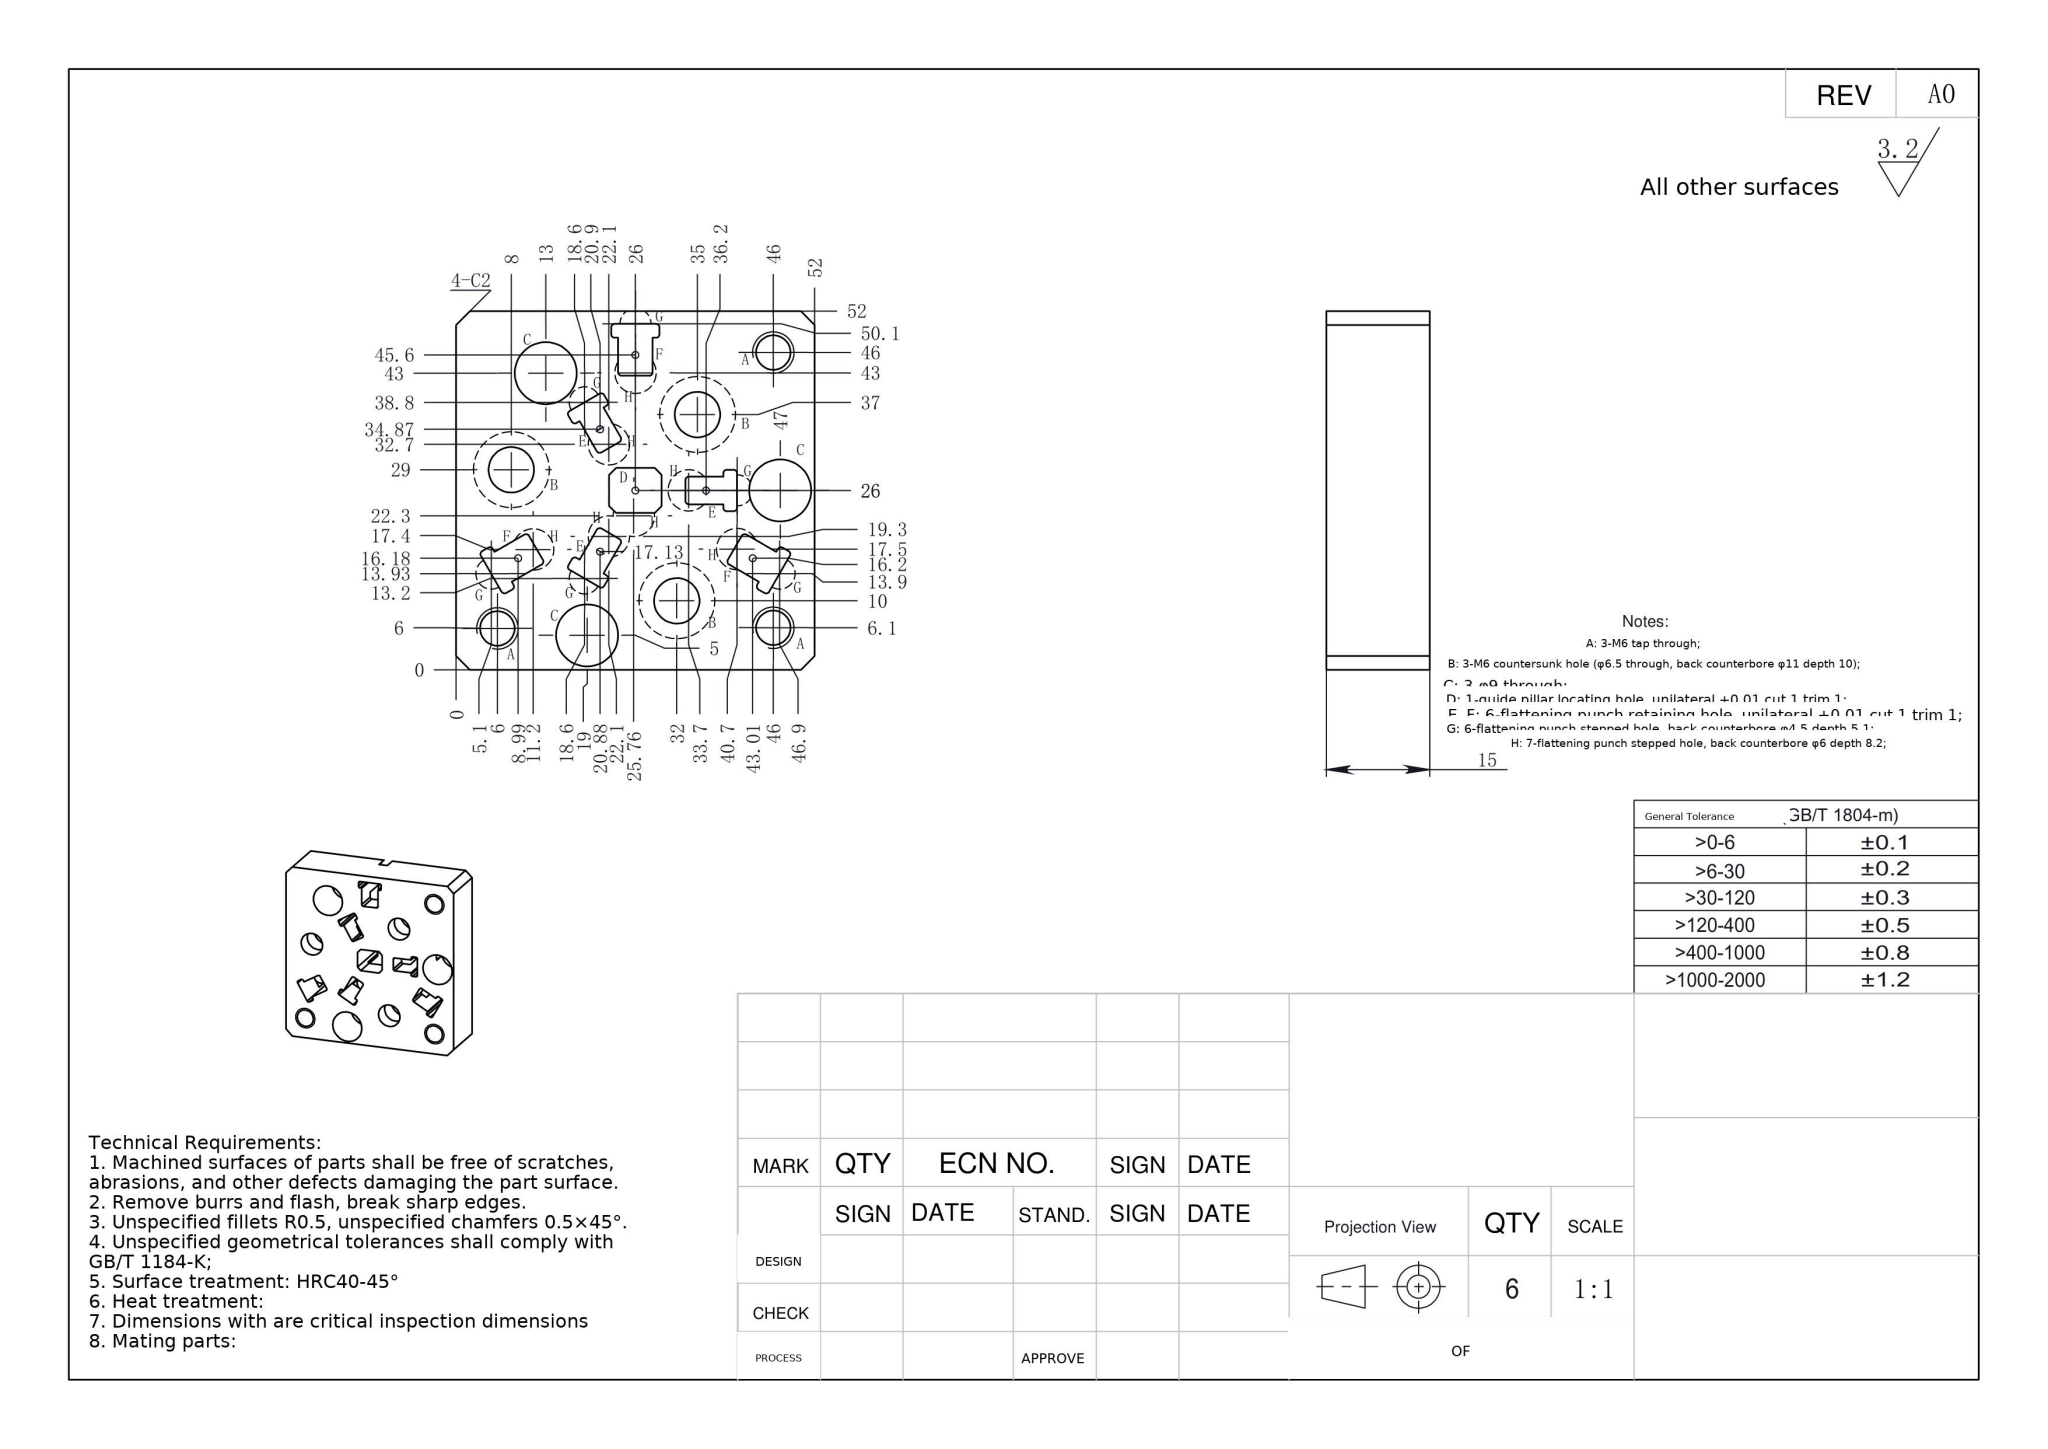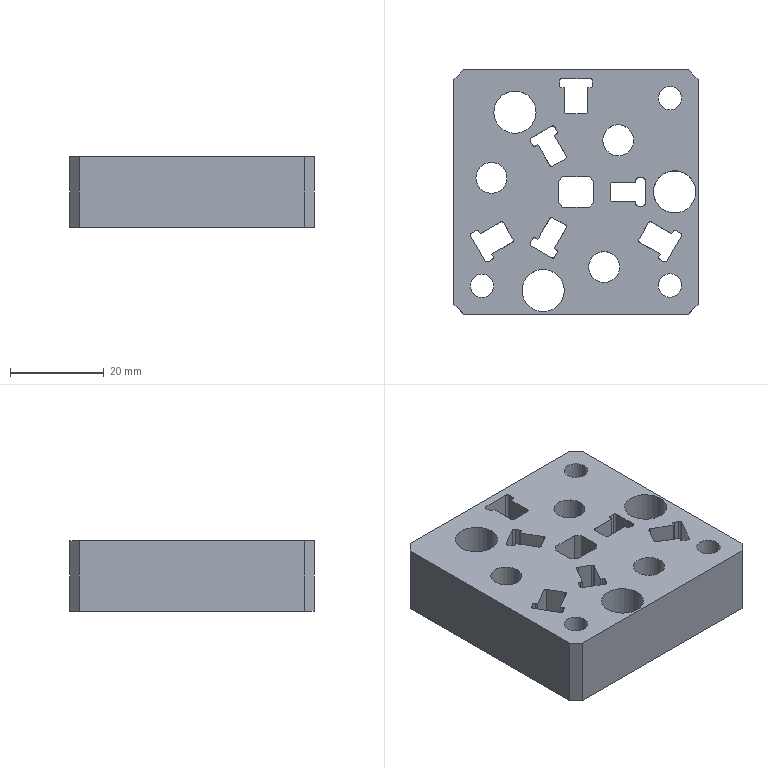Part | SolidWorks | mm | 1 solid | 176 faces | box 52 x 52 x 15 mm | volume 28235 mm3 | cylinder 95 | plane 81 | commonest cylinder face diameters 1 x43 6 x17 4.5 x11 9 x6 5 x6 11 x6 6.6 x6
build123d program:
from build123d import *

# Parameters (mm, degrees)
SKETCH2_W                                            = 52
SKETCH2_H                                            = 52
EXTRUDE1_DEPTH                                       = 15
CBORE_FOR_M6_HEXAGON_SOCKET_HEAD_CAP_SCR_D           = 6.6
CBORE_FOR_M6_HEXAGON_SOCKET_HEAD_CAP_SCR_CBORE_D     = 11
CBORE_FOR_M6_HEXAGON_SOCKET_HEAD_CAP_SCR_CBORE_DEPTH = 10
M6_TAPPED_HOLE1_D                                    = 5
M6_TAPPED_HOLE1_DEPTH                                = 15
M6_TAPPED_HOLE1_TIP                                  = 1.502
SKETCH6_R                                            = 2.05
EXTRUDE3_DEPTH                                       = 6977.79
SKETCH7_R                                            = 4.5
EXTRUDE4_DEPTH                                       = 6977.79
EXTRUDE5_DEPTH                                       = 6977.79
SKETCH9_R                                            = 2.25
EXTRUDE6_DEPTH                                       = 4.2
SKETCH10_R                                           = 3
EXTRUDE7_DEPTH                                       = 8.2
CHAMFER1_SIZE                                        = 2


with BuildPart() as part:
    # Sketch2 → Extrude1 (new body)
    with BuildSketch(Plane.XY):
        with Locations((6481.369, 2489.853)):
            Rectangle(SKETCH2_W, SKETCH2_H)
    extrude(amount=EXTRUDE1_DEPTH)

    # CBORE for M6 Hexagon socket head cap scr (through all)
    with Locations(Plane(origin=(0, 0, 0), x_dir=(-1, 0, 0), z_dir=(0, 0, -1))):
        with Locations((-6490.369, 2500.853), (-6463.369, 2492.853), (-6487.369, 2473.853)):
            CounterBoreHole(CBORE_FOR_M6_HEXAGON_SOCKET_HEAD_CAP_SCR_D / 2, CBORE_FOR_M6_HEXAGON_SOCKET_HEAD_CAP_SCR_CBORE_D / 2, CBORE_FOR_M6_HEXAGON_SOCKET_HEAD_CAP_SCR_CBORE_DEPTH)

    # M6 Tapped Hole1
    with Locations(Plane.XY.offset(15)):
        with Locations((6501.369, 2509.853), (6461.351, 2469.855), (6501.369, 2469.953)):
            Hole(M6_TAPPED_HOLE1_D / 2, depth=M6_TAPPED_HOLE1_DEPTH)
            with Locations((0, 0, -(M6_TAPPED_HOLE1_DEPTH + M6_TAPPED_HOLE1_TIP / 2))):  # 118° drill point
                Cone(0, M6_TAPPED_HOLE1_D / 2, M6_TAPPED_HOLE1_TIP, mode=Mode.SUBTRACT)

    # Sketch6 → Extrude3 (cut, through all)
    with BuildSketch(Plane.XY.offset(15)):
        with Locations((6468.369, 2506.853)):
            Circle(SKETCH6_R)
        with Locations((6474.369, 2468.853)):
            Circle(SKETCH6_R)
        with Locations((6502.369, 2489.853)):
            Circle(SKETCH6_R)
    extrude(amount=-EXTRUDE3_DEPTH, mode=Mode.SUBTRACT)

    # Sketch7 → Extrude4 (cut, through all)
    with BuildSketch(Plane(origin=(0, 0, 0), x_dir=(-1, 0, 0), z_dir=(0, 0, -1))):
        with Locations((-6468.369, 2506.853)):
            Circle(SKETCH7_R)
        with Locations((-6474.369, 2468.853)):
            Circle(SKETCH7_R)
        with Locations((-6502.369, 2489.853)):
            Circle(SKETCH7_R)
    extrude(amount=-EXTRUDE4_DEPTH, mode=Mode.SUBTRACT)

    # Sketch8 → Extrude5 (cut, through all)
    with BuildSketch(Plane.XY.offset(15)):
        with BuildLine():
            Line((6478.869, 2511.996), (6478.369, 2511.996))
            ThreePointArc((6478.369, 2511.996), (6478.016, 2512.142), (6477.869, 2512.496))
            Line((6477.869, 2512.496), (6477.869, 2513.496))
            ThreePointArc((6477.869, 2513.496), (6478.016, 2513.849), (6478.369, 2513.996))
            Line((6478.369, 2513.996), (6484.369, 2513.996))
            ThreePointArc((6484.369, 2513.996), (6484.723, 2513.849), (6484.869, 2513.496))
            Line((6484.869, 2513.496), (6484.869, 2512.496))
            ThreePointArc((6484.869, 2512.496), (6484.723, 2512.142), (6484.369, 2511.996))
            Line((6484.369, 2511.996), (6483.869, 2511.996))
            Line((6483.869, 2511.996), (6483.869, 2506.996))
            ThreePointArc((6483.869, 2506.996), (6483.723, 2506.642), (6483.369, 2506.496))
            Line((6483.369, 2506.496), (6479.369, 2506.496))
            ThreePointArc((6479.369, 2506.496), (6479.016, 2506.642), (6478.869, 2506.996))
            Line((6478.869, 2506.996), (6478.869, 2511.996))
        make_face()
        with BuildLine():
            Line((6479.229, 2497.56), (6476.729, 2501.89))
            Line((6476.729, 2501.89), (6477.162, 2502.14))
            ThreePointArc((6477.162, 2502.14), (6477.395, 2502.444), (6477.345, 2502.823))
            Line((6477.345, 2502.823), (6476.845, 2503.689))
            ThreePointArc((6476.845, 2503.689), (6476.542, 2503.922), (6476.162, 2503.872))
            Line((6476.162, 2503.872), (6471.832, 2501.372))
            ThreePointArc((6471.832, 2501.372), (6471.599, 2501.069), (6471.649, 2500.689))
            Line((6471.649, 2500.689), (6472.149, 2499.823))
            ThreePointArc((6472.149, 2499.823), (6472.453, 2499.59), (6472.832, 2499.64))
            Line((6472.832, 2499.64), (6473.265, 2499.89))
            Line((6473.265, 2499.89), (6475.765, 2495.56))
            ThreePointArc((6475.765, 2495.56), (6476.069, 2495.327), (6476.448, 2495.377))
            Line((6476.448, 2495.377), (6479.046, 2496.877))
            ThreePointArc((6479.046, 2496.877), (6479.279, 2497.181), (6479.229, 2497.56))
        make_face()
        with BuildLine():
            Line((6488.614, 2491.353), (6488.614, 2488.353))
            ThreePointArc((6488.614, 2488.353), (6488.76, 2488), (6489.114, 2487.853))
            Line((6489.114, 2487.853), (6494.114, 2487.853))
            Line((6494.114, 2487.853), (6494.114, 2487.353))
            ThreePointArc((6494.114, 2487.353), (6494.26, 2487), (6494.614, 2486.853))
            Line((6494.614, 2486.853), (6495.614, 2486.853))
            ThreePointArc((6495.614, 2486.853), (6495.968, 2487), (6496.114, 2487.353))
            Line((6496.114, 2487.353), (6496.114, 2492.353))
            ThreePointArc((6496.114, 2492.353), (6495.968, 2492.707), (6495.614, 2492.853))
            Line((6495.614, 2492.853), (6494.614, 2492.853))
            ThreePointArc((6494.614, 2492.853), (6494.26, 2492.707), (6494.114, 2492.353))
            Line((6494.114, 2492.353), (6494.114, 2491.853))
            Line((6494.114, 2491.853), (6489.114, 2491.853))
            ThreePointArc((6489.114, 2491.853), (6488.76, 2491.707), (6488.614, 2491.353))
        make_face()
        with BuildLine():
            Line((6499.295, 2476.617), (6494.965, 2479.117))
            ThreePointArc((6494.965, 2479.117), (6494.732, 2479.421), (6494.782, 2479.8))
            Line((6494.782, 2479.8), (6496.782, 2483.264))
            ThreePointArc((6496.782, 2483.264), (6497.086, 2483.497), (6497.465, 2483.447))
            Line((6497.465, 2483.447), (6501.795, 2480.947))
            Line((6501.795, 2480.947), (6502.045, 2481.38))
            ThreePointArc((6502.045, 2481.38), (6502.349, 2481.613), (6502.728, 2481.563))
            Line((6502.728, 2481.563), (6503.594, 2481.063))
            ThreePointArc((6503.594, 2481.063), (6503.827, 2480.76), (6503.777, 2480.38))
            Line((6503.777, 2480.38), (6500.777, 2475.184))
            ThreePointArc((6500.777, 2475.184), (6500.474, 2474.951), (6500.094, 2475.001))
            Line((6500.094, 2475.001), (6499.228, 2475.501))
            ThreePointArc((6499.228, 2475.501), (6498.995, 2475.805), (6499.045, 2476.184))
            Line((6499.045, 2476.184), (6499.295, 2476.617))
        make_face()
        with BuildLine():
            Line((6475.765, 2484.146), (6473.265, 2479.816))
            Line((6473.265, 2479.816), (6472.832, 2480.066))
            ThreePointArc((6472.832, 2480.066), (6472.453, 2480.116), (6472.149, 2479.883))
            Line((6472.149, 2479.883), (6471.649, 2479.017))
            ThreePointArc((6471.649, 2479.017), (6471.599, 2478.638), (6471.832, 2478.334))
            Line((6471.832, 2478.334), (6476.162, 2475.834))
            ThreePointArc((6476.162, 2475.834), (6476.542, 2475.784), (6476.845, 2476.017))
            Line((6476.845, 2476.017), (6477.345, 2476.883))
            ThreePointArc((6477.345, 2476.883), (6477.395, 2477.263), (6477.162, 2477.566))
            Line((6477.162, 2477.566), (6476.729, 2477.816))
            Line((6476.729, 2477.816), (6479.229, 2482.146))
            ThreePointArc((6479.229, 2482.146), (6479.279, 2482.526), (6479.046, 2482.829))
            Line((6479.046, 2482.829), (6476.448, 2484.329))
            ThreePointArc((6476.448, 2484.329), (6476.069, 2484.379), (6475.765, 2484.146))
        make_face()
        with BuildLine():
            Line((6458.962, 2480.38), (6461.962, 2475.184))
            ThreePointArc((6461.962, 2475.184), (6462.265, 2474.951), (6462.645, 2475.001))
            Line((6462.645, 2475.001), (6463.511, 2475.501))
            ThreePointArc((6463.511, 2475.501), (6463.744, 2475.805), (6463.694, 2476.184))
            Line((6463.694, 2476.184), (6463.444, 2476.617))
            Line((6463.444, 2476.617), (6467.774, 2479.117))
            ThreePointArc((6467.774, 2479.117), (6468.007, 2479.421), (6467.957, 2479.8))
            Line((6467.957, 2479.8), (6465.957, 2483.264))
            ThreePointArc((6465.957, 2483.264), (6465.653, 2483.497), (6465.274, 2483.447))
            Line((6465.274, 2483.447), (6460.944, 2480.947))
            Line((6460.944, 2480.947), (6460.694, 2481.38))
            ThreePointArc((6460.694, 2481.38), (6460.39, 2481.613), (6460.011, 2481.563))
            Line((6460.011, 2481.563), (6459.145, 2481.063))
            ThreePointArc((6459.145, 2481.063), (6458.912, 2480.76), (6458.962, 2480.38))
        make_face()
        Polygon((6477.559, 2492.113), (6478.559, 2493.113), (6484.179, 2493.113), (6485.179, 2492.113), (6485.179, 2487.593), (6484.179, 2486.593), (6478.559, 2486.593), (6477.559, 2487.593), align=None)
    extrude(amount=-EXTRUDE5_DEPTH, mode=Mode.SUBTRACT)

    # Sketch9 → Extrude6 (cut)
    with BuildSketch(Plane(origin=(0, 0, 0), x_dir=(-1, 0, 0), z_dir=(0, 0, -1))):
        with Locations((-6473.997, 2502.622)):
            Circle(SKETCH9_R)
        with Locations((-6481.369, 2513.996)):
            Circle(SKETCH9_R)
        with Locations((-6502.277, 2477.782)):
            Circle(SKETCH9_R)
        with Locations((-6473.997, 2477.084)):
            Circle(SKETCH9_R)
        with Locations((-6460.462, 2477.782)):
            Circle(SKETCH9_R)
        with Locations((-6496.114, 2489.853)):
            Circle(SKETCH9_R)
    extrude(amount=-EXTRUDE6_DEPTH, mode=Mode.SUBTRACT)

    # Sketch10 → Extrude7 (cut)
    with BuildSketch(Plane(origin=(0, 0, 0), x_dir=(-1, 0, 0), z_dir=(0, 0, -1))):
        with Locations((-6481.369, 2506.896)):
            Circle(SKETCH10_R)
        with Locations((-6477.511, 2496.537)):
            Circle(SKETCH10_R)
        with Locations((-6466.529, 2481.285)):
            Circle(SKETCH10_R)
        with Locations((-6496.108, 2481.344)):
            Circle(SKETCH10_R)
        with Locations((-6489.087, 2489.853)):
            Circle(SKETCH10_R)
        with BuildLine():
            ThreePointArc((-6478.126, 2486.106), (-6483.436, 2488.076), (-6480.51, 2483.226))
            ThreePointArc((-6480.51, 2483.226), (-6475.2, 2481.257), (-6478.126, 2486.106))
        make_face()
    extrude(amount=-EXTRUDE7_DEPTH, mode=Mode.SUBTRACT)

    # Chamfer1
    chamfer1_edges = [part.edges().sort_by_distance(p)[0] for p in [
        (6507.369, 2463.853, 7.5),
        (6455.369, 2463.853, 7.5),
        (6455.369, 2515.853, 7.5),
        (6507.369, 2515.853, 7.5),
    ]]
    chamfer(chamfer1_edges, length=CHAMFER1_SIZE)


solid = part.part